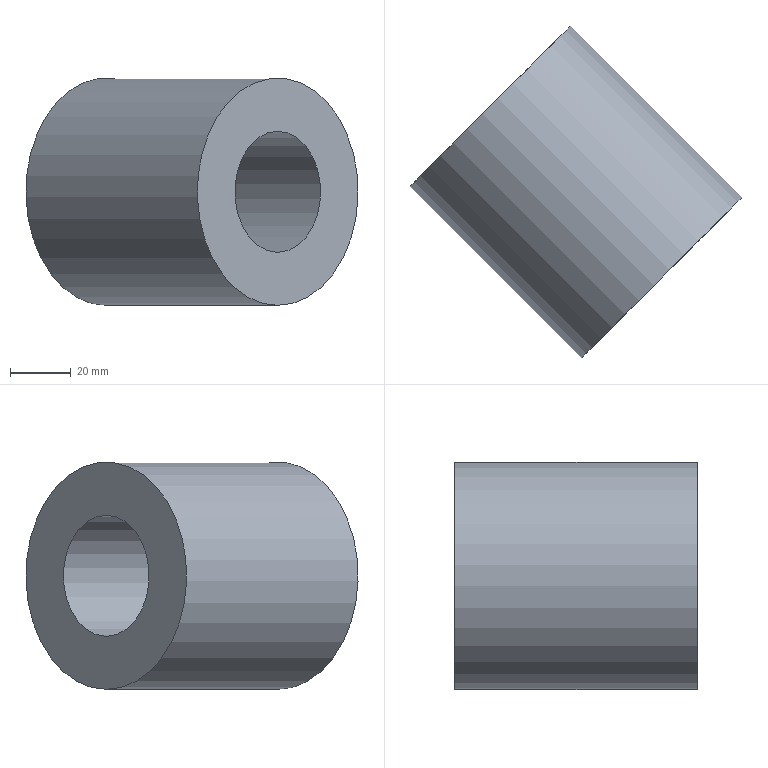Component | NX | SLID_FRAME_SLID_RING_2 | 1 solid | 4 faces | box 109.6 x 109.6 x 75 mm | volume 252898 mm3 | cylinder 2 | plane 2 | commonest cylinder face diameters 75 x1 40 x1
STEP:
#1=CARTESIAN_POINT('',(0.,0.,0.));
#2=DIRECTION('',(0.,0.,1.));
#3=DIRECTION('',(1.,0.,0.));
#4=AXIS2_PLACEMENT_3D('',#1,#2,#3);
#5=CARTESIAN_POINT('',(-700.456,706.902,422.5));
#6=VERTEX_POINT('',#5);
#7=CARTESIAN_POINT('',(-700.456,706.902,460.));
#8=DIRECTION('',(0.7071,-0.7071,0.));
#9=DIRECTION('',(0.,0.,-1.));
#10=AXIS2_PLACEMENT_3D('',#7,#8,#9);
#11=CIRCLE('',#10,37.5);
#12=CARTESIAN_POINT('',(-700.456,706.902,460.));
#13=DIRECTION('',(0.7071,-0.7071,0.));
#14=DIRECTION('',(0.,0.,1.));
#15=AXIS2_PLACEMENT_3D('',#12,#13,#14);
#16=CYLINDRICAL_SURFACE('',#15,37.5);
#17=CARTESIAN_POINT('',(3.142,0.));
#18=DIRECTION('',(1.,0.));
#19=VECTOR('',#18,1.);
#20=LINE('',#17,#19);
#21=(GEOMETRIC_REPRESENTATION_CONTEXT(2)PARAMETRIC_REPRESENTATION_CONTEXT()REPRESENTATION_CONTEXT('',''));
#22=DEFINITIONAL_REPRESENTATION('',(#20),#21);
#23=PCURVE('',#16,#22);
#24=CARTESIAN_POINT('',(-700.456,706.902,460.));
#25=DIRECTION('',(0.7071,-0.7071,0.));
#26=DIRECTION('',(0.,0.,1.));
#27=AXIS2_PLACEMENT_3D('',#24,#25,#26);
#28=PLANE('',#27);
#29=CARTESIAN_POINT('',(0.,0.));
#30=DIRECTION('',(-1.,0.));
#31=AXIS2_PLACEMENT_2D('',#29,#30);
#32=CIRCLE('',#31,37.5);
#33=(GEOMETRIC_REPRESENTATION_CONTEXT(2)PARAMETRIC_REPRESENTATION_CONTEXT()REPRESENTATION_CONTEXT('',''));
#34=DEFINITIONAL_REPRESENTATION('',(#32),#33);
#35=PCURVE('',#28,#34);
#36=SURFACE_CURVE('',#11,(#23,#35),.PCURVE_S1.);
#37=EDGE_CURVE('',#6,#6,#36,.T.);
#38=ORIENTED_EDGE('',*,*,#37,.T.);
#39=CARTESIAN_POINT('',(-643.888,650.334,422.5));
#40=VERTEX_POINT('',#39);
#41=CARTESIAN_POINT('',(-700.456,706.902,422.5));
#42=CARTESIAN_POINT('',(-643.888,650.334,422.5));
#43=B_SPLINE_CURVE_WITH_KNOTS('',1,(#41,#42),.UNSPECIFIED.,.F.,.F.,(2,2),(0.,80.),.PIECEWISE_BEZIER_KNOTS.);
#44=CARTESIAN_POINT('',(9.425,0.));
#45=DIRECTION('',(0.,1.));
#46=VECTOR('',#45,1.);
#47=LINE('',#44,#46);
#48=(GEOMETRIC_REPRESENTATION_CONTEXT(2)PARAMETRIC_REPRESENTATION_CONTEXT()REPRESENTATION_CONTEXT('',''));
#49=DEFINITIONAL_REPRESENTATION('',(#47),#48);
#50=PCURVE('',#16,#49);
#51=CARTESIAN_POINT('',(3.142,0.));
#52=DIRECTION('',(0.,1.));
#53=VECTOR('',#52,1.);
#54=LINE('',#51,#53);
#55=(GEOMETRIC_REPRESENTATION_CONTEXT(2)PARAMETRIC_REPRESENTATION_CONTEXT()REPRESENTATION_CONTEXT('',''));
#56=DEFINITIONAL_REPRESENTATION('',(#54),#55);
#57=PCURVE('',#16,#56);
#58=SEAM_CURVE('',#43,(#50,#57),.PCURVE_S1.);
#59=EDGE_CURVE('',#6,#40,#58,.T.);
#60=ORIENTED_EDGE('',*,*,#59,.T.);
#61=CARTESIAN_POINT('',(-643.888,650.334,460.));
#62=DIRECTION('',(0.7071,-0.7071,0.));
#63=DIRECTION('',(0.,0.,-1.));
#64=AXIS2_PLACEMENT_3D('',#61,#62,#63);
#65=CIRCLE('',#64,37.5);
#66=CARTESIAN_POINT('',(3.142,80.));
#67=DIRECTION('',(1.,0.));
#68=VECTOR('',#67,1.);
#69=LINE('',#66,#68);
#70=(GEOMETRIC_REPRESENTATION_CONTEXT(2)PARAMETRIC_REPRESENTATION_CONTEXT()REPRESENTATION_CONTEXT('',''));
#71=DEFINITIONAL_REPRESENTATION('',(#69),#70);
#72=PCURVE('',#16,#71);
#73=CARTESIAN_POINT('',(-643.888,650.334,460.));
#74=DIRECTION('',(0.7071,-0.7071,0.));
#75=DIRECTION('',(0.,0.,1.));
#76=AXIS2_PLACEMENT_3D('',#73,#74,#75);
#77=PLANE('',#76);
#78=CARTESIAN_POINT('',(0.,0.));
#79=DIRECTION('',(-1.,0.));
#80=AXIS2_PLACEMENT_2D('',#78,#79);
#81=CIRCLE('',#80,37.5);
#82=(GEOMETRIC_REPRESENTATION_CONTEXT(2)PARAMETRIC_REPRESENTATION_CONTEXT()REPRESENTATION_CONTEXT('',''));
#83=DEFINITIONAL_REPRESENTATION('',(#81),#82);
#84=PCURVE('',#77,#83);
#85=SURFACE_CURVE('',#65,(#72,#84),.PCURVE_S1.);
#86=EDGE_CURVE('',#40,#40,#85,.T.);
#87=ORIENTED_EDGE('',*,*,#86,.F.);
#88=ORIENTED_EDGE('',*,*,#59,.F.);
#89=EDGE_LOOP('',(#38,#60,#87,#88));
#90=FACE_BOUND('',#89,.T.);
#91=ADVANCED_FACE('',(#90),#16,.T.);
#92=CARTESIAN_POINT('',(-700.456,706.902,440.));
#93=VERTEX_POINT('',#92);
#94=CARTESIAN_POINT('',(-700.456,706.902,460.));
#95=DIRECTION('',(0.7071,-0.7071,0.));
#96=DIRECTION('',(0.,0.,-1.));
#97=AXIS2_PLACEMENT_3D('',#94,#95,#96);
#98=CIRCLE('',#97,20.);
#99=CARTESIAN_POINT('',(-700.456,706.902,460.));
#100=DIRECTION('',(0.7071,-0.7071,0.));
#101=DIRECTION('',(0.,0.,1.));
#102=AXIS2_PLACEMENT_3D('',#99,#100,#101);
#103=CYLINDRICAL_SURFACE('',#102,20.);
#104=CARTESIAN_POINT('',(3.142,0.));
#105=DIRECTION('',(1.,0.));
#106=VECTOR('',#105,1.);
#107=LINE('',#104,#106);
#108=(GEOMETRIC_REPRESENTATION_CONTEXT(2)PARAMETRIC_REPRESENTATION_CONTEXT()REPRESENTATION_CONTEXT('',''));
#109=DEFINITIONAL_REPRESENTATION('',(#107),#108);
#110=PCURVE('',#103,#109);
#111=CARTESIAN_POINT('',(0.,0.));
#112=DIRECTION('',(-1.,0.));
#113=AXIS2_PLACEMENT_2D('',#111,#112);
#114=CIRCLE('',#113,20.);
#115=(GEOMETRIC_REPRESENTATION_CONTEXT(2)PARAMETRIC_REPRESENTATION_CONTEXT()REPRESENTATION_CONTEXT('',''));
#116=DEFINITIONAL_REPRESENTATION('',(#114),#115);
#117=PCURVE('',#28,#116);
#118=SURFACE_CURVE('',#98,(#110,#117),.PCURVE_S1.);
#119=EDGE_CURVE('',#93,#93,#118,.T.);
#120=ORIENTED_EDGE('',*,*,#119,.T.);
#121=CARTESIAN_POINT('',(-643.888,650.334,440.));
#122=VERTEX_POINT('',#121);
#123=CARTESIAN_POINT('',(-700.456,706.902,440.));
#124=CARTESIAN_POINT('',(-643.888,650.334,440.));
#125=B_SPLINE_CURVE_WITH_KNOTS('',1,(#123,#124),.UNSPECIFIED.,.F.,.F.,(2,2),(0.,80.),.PIECEWISE_BEZIER_KNOTS.);
#126=CARTESIAN_POINT('',(9.425,0.));
#127=DIRECTION('',(0.,1.));
#128=VECTOR('',#127,1.);
#129=LINE('',#126,#128);
#130=(GEOMETRIC_REPRESENTATION_CONTEXT(2)PARAMETRIC_REPRESENTATION_CONTEXT()REPRESENTATION_CONTEXT('',''));
#131=DEFINITIONAL_REPRESENTATION('',(#129),#130);
#132=PCURVE('',#103,#131);
#133=CARTESIAN_POINT('',(3.142,0.));
#134=DIRECTION('',(0.,1.));
#135=VECTOR('',#134,1.);
#136=LINE('',#133,#135);
#137=(GEOMETRIC_REPRESENTATION_CONTEXT(2)PARAMETRIC_REPRESENTATION_CONTEXT()REPRESENTATION_CONTEXT('',''));
#138=DEFINITIONAL_REPRESENTATION('',(#136),#137);
#139=PCURVE('',#103,#138);
#140=SEAM_CURVE('',#125,(#132,#139),.PCURVE_S1.);
#141=EDGE_CURVE('',#93,#122,#140,.T.);
#142=ORIENTED_EDGE('',*,*,#141,.T.);
#143=CARTESIAN_POINT('',(-643.888,650.334,460.));
#144=DIRECTION('',(0.7071,-0.7071,0.));
#145=DIRECTION('',(0.,0.,-1.));
#146=AXIS2_PLACEMENT_3D('',#143,#144,#145);
#147=CIRCLE('',#146,20.);
#148=CARTESIAN_POINT('',(3.142,80.));
#149=DIRECTION('',(1.,0.));
#150=VECTOR('',#149,1.);
#151=LINE('',#148,#150);
#152=(GEOMETRIC_REPRESENTATION_CONTEXT(2)PARAMETRIC_REPRESENTATION_CONTEXT()REPRESENTATION_CONTEXT('',''));
#153=DEFINITIONAL_REPRESENTATION('',(#151),#152);
#154=PCURVE('',#103,#153);
#155=CARTESIAN_POINT('',(0.,0.));
#156=DIRECTION('',(-1.,0.));
#157=AXIS2_PLACEMENT_2D('',#155,#156);
#158=CIRCLE('',#157,20.);
#159=(GEOMETRIC_REPRESENTATION_CONTEXT(2)PARAMETRIC_REPRESENTATION_CONTEXT()REPRESENTATION_CONTEXT('',''));
#160=DEFINITIONAL_REPRESENTATION('',(#158),#159);
#161=PCURVE('',#77,#160);
#162=SURFACE_CURVE('',#147,(#154,#161),.PCURVE_S1.);
#163=EDGE_CURVE('',#122,#122,#162,.T.);
#164=ORIENTED_EDGE('',*,*,#163,.F.);
#165=ORIENTED_EDGE('',*,*,#141,.F.);
#166=EDGE_LOOP('',(#120,#142,#164,#165));
#167=FACE_BOUND('',#166,.F.);
#168=ADVANCED_FACE('',(#167),#103,.F.);
#169=ORIENTED_EDGE('',*,*,#37,.F.);
#170=EDGE_LOOP('',(#169));
#171=FACE_BOUND('',#170,.T.);
#172=ORIENTED_EDGE('',*,*,#119,.T.);
#173=EDGE_LOOP('',(#172));
#174=FACE_BOUND('',#173,.T.);
#175=ADVANCED_FACE('',(#171,#174),#28,.F.);
#176=ORIENTED_EDGE('',*,*,#86,.T.);
#177=EDGE_LOOP('',(#176));
#178=FACE_BOUND('',#177,.T.);
#179=ORIENTED_EDGE('',*,*,#163,.F.);
#180=EDGE_LOOP('',(#179));
#181=FACE_BOUND('',#180,.T.);
#182=ADVANCED_FACE('',(#178,#181),#77,.T.);
#183=CLOSED_SHELL('',(#91,#168,#175,#182));
#184=MANIFOLD_SOLID_BREP('',#183);
#185=(LENGTH_UNIT()NAMED_UNIT(*)SI_UNIT(.MILLI.,.METRE.));
#186=UNCERTAINTY_MEASURE_WITH_UNIT(LENGTH_MEASURE(0.00001),#185,'','');
#187=(NAMED_UNIT(*)PLANE_ANGLE_UNIT()SI_UNIT($,.RADIAN.));
#188=(NAMED_UNIT(*)SI_UNIT($,.STERADIAN.)SOLID_ANGLE_UNIT());
#189=(GEOMETRIC_REPRESENTATION_CONTEXT(3)GLOBAL_UNCERTAINTY_ASSIGNED_CONTEXT((#186))GLOBAL_UNIT_ASSIGNED_CONTEXT((#185,#187,#188))REPRESENTATION_CONTEXT('',''));
#190=ADVANCED_BREP_SHAPE_REPRESENTATION('',(#4,#184),#189);